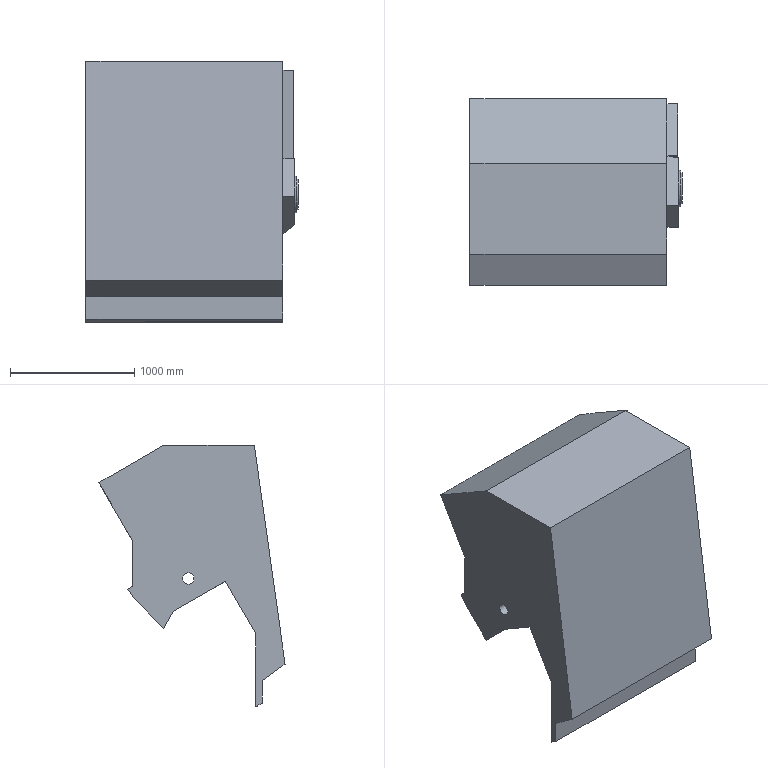Component | NX | SIM15_HAUPTSPINDELSEITE | 1 solid | 61 faces | volume 2441104871 mm3 | plane 54 | cylinder 7 | commonest cylinder face diameters 130 x2 156 x1 295 x1 250 x1 90 x1 770 x1